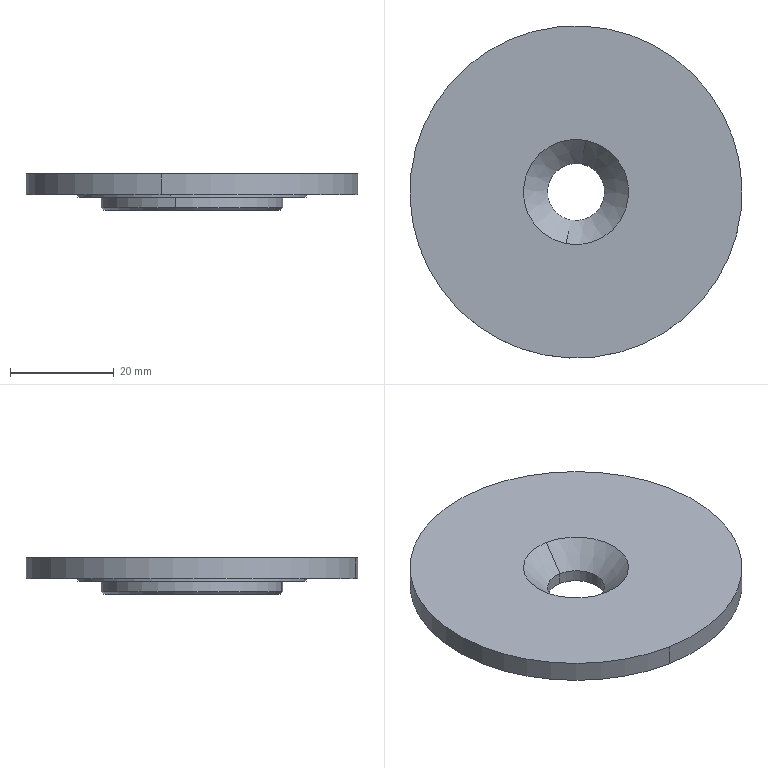Component | SolidWorks | 12AFixedFlatGrooveLargeWheel-EngravingAndMillingAxis-2_12ALargeStraighteningWheelCover-1 | 1 solid | 16 faces | box 64 x 64 x 7 mm | volume 14876 mm3 | cylinder 8 | cone 4 | plane 4 | commonest cylinder face diameters 11 x2 64 x2 44 x2 35 x2 | material 45
build123d program:
from build123d import *

# Parameters (mm, degrees)
HOLE_SIZE_ACCORDING_TO_HEXAGON_SOCKET_D           = 11
HOLE_SIZE_ACCORDING_TO_HEXAGON_SOCKET_DEPTH       = 32.75
HOLE_SIZE_ACCORDING_TO_HEXAGON_SOCKET_CSINK_D     = 20.3
HOLE_SIZE_ACCORDING_TO_HEXAGON_SOCKET_CSINK_ANGLE = 90
HOLE_SIZE_ACCORDING_TO_HEXAGON_SOCKET_TIP         = 3.305
CHAMFER1_SIZE                                     = 0.5


with BuildPart() as part:
    # Sketch1 → Revolve1 (revolve)
    with BuildSketch(Plane.XY, mode=Mode.PRIVATE) as revolve1_sk:
        Polygon((0, 0), (0, 17.5), (2.5, 17.5), (2.5, 22), (3, 22), (3, 32), (7, 32), (7, 0), align=None)
    revolve(revolve1_sk.sketch.rotate(Axis((0, 0, 0), (1, 0, 0)), 90), axis=Axis((0, 0, 0), (1, 0, 0)))

    # Hole Size _ according to_ Hexagon Socket
    with Locations(Plane(origin=(7, 0, 0), x_dir=(0, 0, -1), z_dir=(1, 0, 0))):
        with Locations((0, 0)):
            CounterSinkHole(HOLE_SIZE_ACCORDING_TO_HEXAGON_SOCKET_D / 2, HOLE_SIZE_ACCORDING_TO_HEXAGON_SOCKET_CSINK_D / 2, depth=HOLE_SIZE_ACCORDING_TO_HEXAGON_SOCKET_DEPTH, counter_sink_angle=HOLE_SIZE_ACCORDING_TO_HEXAGON_SOCKET_CSINK_ANGLE)
            with Locations((0, 0, -(HOLE_SIZE_ACCORDING_TO_HEXAGON_SOCKET_DEPTH + HOLE_SIZE_ACCORDING_TO_HEXAGON_SOCKET_TIP / 2))):  # 118° drill point
                Cone(0, HOLE_SIZE_ACCORDING_TO_HEXAGON_SOCKET_D / 2, HOLE_SIZE_ACCORDING_TO_HEXAGON_SOCKET_TIP, mode=Mode.SUBTRACT)

    # Chamfer1
    chamfer1_edges = [part.edges().sort_by_distance(p)[0] for p in [
        (0, 0, -17.5),
    ]]
    chamfer(chamfer1_edges, length=CHAMFER1_SIZE)


solid = part.part

# Placed as in the assembly
solid = solid.moved(Location((-257.402, 59.038, 49.25), (0, -90, 0)))
STEP:
#1=COLOUR_RGB('',0.7922,0.8196,0.9333);
#2=FILL_AREA_STYLE_COLOUR('',#1);
#3=FILL_AREA_STYLE('',(#2));
#4=SURFACE_STYLE_FILL_AREA(#3);
#5=SURFACE_SIDE_STYLE('',(#4));
#6=SURFACE_STYLE_USAGE(.BOTH.,#5);
#7=PRESENTATION_STYLE_ASSIGNMENT((#6));
#8=CARTESIAN_POINT('',(-10.259,1.667,1.939));
#9=VERTEX_POINT('',#8);
#10=CARTESIAN_POINT('',(-10.009,2.982,1.939));
#11=VERTEX_POINT('',#10);
#12=CARTESIAN_POINT('',(-10.134,2.324,1.939));
#13=DIRECTION('',(-0.,0.,-1.));
#14=DIRECTION('',(0.1862,0.9825,0.));
#15=AXIS2_PLACEMENT_3D('',#12,#13,#14);
#16=CIRCLE('',#15,0.6693);
#17=EDGE_CURVE('',#9,#11,#16,.T.);
#18=ORIENTED_EDGE('',*,*,#17,.F.);
#19=CARTESIAN_POINT('',(-10.262,1.647,1.959));
#20=VERTEX_POINT('',#19);
#21=CARTESIAN_POINT('',(-10.259,1.667,1.939));
#22=DIRECTION('',(-0.1316,-0.6947,0.7071));
#23=VECTOR('',#22,39.37);
#24=LINE('',#21,#23);
#25=EDGE_CURVE('',#9,#20,#24,.T.);
#26=ORIENTED_EDGE('',*,*,#25,.T.);
#27=CARTESIAN_POINT('',(-10.006,3.001,1.959));
#28=VERTEX_POINT('',#27);
#29=CARTESIAN_POINT('',(-10.134,2.324,1.959));
#30=DIRECTION('',(0.,-0.,1.));
#31=DIRECTION('',(0.1862,0.9825,0.));
#32=AXIS2_PLACEMENT_3D('',#29,#30,#31);
#33=CIRCLE('',#32,0.689);
#34=EDGE_CURVE('',#28,#20,#33,.T.);
#35=ORIENTED_EDGE('',*,*,#34,.F.);
#36=CARTESIAN_POINT('',(-10.009,2.982,1.939));
#37=DIRECTION('',(0.1316,0.6947,0.7071));
#38=VECTOR('',#37,39.37);
#39=LINE('',#36,#38);
#40=EDGE_CURVE('',#11,#28,#39,.T.);
#41=ORIENTED_EDGE('',*,*,#40,.F.);
#42=EDGE_LOOP('',(#18,#26,#35,#41));
#43=FACE_OUTER_BOUND('',#42,.T.);
#44=CARTESIAN_POINT('',(-10.134,2.324,1.939));
#45=DIRECTION('',(0.,-0.,1.));
#46=DIRECTION('',(0.1862,0.9825,0.));
#47=AXIS2_PLACEMENT_3D('',#44,#45,#46);
#48=CONICAL_SURFACE('',#47,0.6693,0.7854);
#49=ADVANCED_FACE('',(#43),#48,.T.);
#50=CARTESIAN_POINT('',(-10.174,2.112,2.031));
#51=VERTEX_POINT('',#50);
#52=CARTESIAN_POINT('',(-10.094,2.537,2.031));
#53=VERTEX_POINT('',#52);
#54=CARTESIAN_POINT('',(-10.134,2.324,2.031));
#55=DIRECTION('',(0.,-0.,1.));
#56=DIRECTION('',(0.1862,0.9825,0.));
#57=AXIS2_PLACEMENT_3D('',#54,#55,#56);
#58=CIRCLE('',#57,0.2165);
#59=EDGE_CURVE('',#51,#53,#58,.T.);
#60=ORIENTED_EDGE('',*,*,#59,.F.);
#61=CARTESIAN_POINT('',(-10.208,1.932,2.215));
#62=VERTEX_POINT('',#61);
#63=CARTESIAN_POINT('',(-10.208,1.932,2.215));
#64=DIRECTION('',(-0.1316,-0.6947,0.7071));
#65=VECTOR('',#64,39.37);
#66=LINE('',#63,#65);
#67=EDGE_CURVE('',#51,#62,#66,.T.);
#68=ORIENTED_EDGE('',*,*,#67,.T.);
#69=CARTESIAN_POINT('',(-10.06,2.717,2.215));
#70=VERTEX_POINT('',#69);
#71=CARTESIAN_POINT('',(-10.134,2.324,2.215));
#72=DIRECTION('',(0.,-0.,1.));
#73=DIRECTION('',(0.1862,0.9825,0.));
#74=AXIS2_PLACEMENT_3D('',#71,#72,#73);
#75=CIRCLE('',#74,0.3996);
#76=EDGE_CURVE('',#62,#70,#75,.T.);
#77=ORIENTED_EDGE('',*,*,#76,.T.);
#78=CARTESIAN_POINT('',(-10.06,2.717,2.215));
#79=DIRECTION('',(0.1316,0.6947,0.7071));
#80=VECTOR('',#79,39.37);
#81=LINE('',#78,#80);
#82=EDGE_CURVE('',#53,#70,#81,.T.);
#83=ORIENTED_EDGE('',*,*,#82,.F.);
#84=EDGE_LOOP('',(#60,#68,#77,#83));
#85=FACE_OUTER_BOUND('',#84,.T.);
#86=CARTESIAN_POINT('',(-10.134,2.324,2.215));
#87=DIRECTION('',(0.,-0.,1.));
#88=DIRECTION('',(0.1862,0.9825,0.));
#89=AXIS2_PLACEMENT_3D('',#86,#87,#88);
#90=CONICAL_SURFACE('',#89,0.3996,0.7854);
#91=ADVANCED_FACE('',(#85),#90,.F.);
#92=CARTESIAN_POINT('',(-10.174,2.112,1.939));
#93=VERTEX_POINT('',#92);
#94=CARTESIAN_POINT('',(-10.094,2.537,1.939));
#95=VERTEX_POINT('',#94);
#96=CARTESIAN_POINT('',(-10.134,2.324,1.939));
#97=DIRECTION('',(0.,-0.,1.));
#98=DIRECTION('',(0.1862,0.9825,0.));
#99=AXIS2_PLACEMENT_3D('',#96,#97,#98);
#100=CIRCLE('',#99,0.2165);
#101=EDGE_CURVE('',#93,#95,#100,.T.);
#102=ORIENTED_EDGE('',*,*,#101,.F.);
#103=CARTESIAN_POINT('',(-10.174,2.112,2.215));
#104=DIRECTION('',(0.,-0.,1.));
#105=VECTOR('',#104,39.37);
#106=LINE('',#103,#105);
#107=EDGE_CURVE('',#93,#51,#106,.T.);
#108=ORIENTED_EDGE('',*,*,#107,.T.);
#109=ORIENTED_EDGE('',*,*,#59,.T.);
#110=CARTESIAN_POINT('',(-10.094,2.537,2.215));
#111=DIRECTION('',(0.,-0.,1.));
#112=VECTOR('',#111,39.37);
#113=LINE('',#110,#112);
#114=EDGE_CURVE('',#95,#53,#113,.T.);
#115=ORIENTED_EDGE('',*,*,#114,.F.);
#116=EDGE_LOOP('',(#102,#108,#109,#115));
#117=FACE_OUTER_BOUND('',#116,.T.);
#118=CARTESIAN_POINT('',(-10.134,2.324,2.215));
#119=DIRECTION('',(0.,-0.,1.));
#120=DIRECTION('',(0.1862,0.9825,0.));
#121=AXIS2_PLACEMENT_3D('',#118,#119,#120);
#122=CYLINDRICAL_SURFACE('',#121,0.2165);
#123=ADVANCED_FACE('',(#117),#122,.F.);
#124=CARTESIAN_POINT('',(-10.368,1.087,2.215));
#125=VERTEX_POINT('',#124);
#126=CARTESIAN_POINT('',(-9.899,3.562,2.215));
#127=VERTEX_POINT('',#126);
#128=CARTESIAN_POINT('',(-10.134,2.324,2.215));
#129=DIRECTION('',(-0.,0.,-1.));
#130=DIRECTION('',(-0.1862,-0.9825,0.));
#131=AXIS2_PLACEMENT_3D('',#128,#129,#130);
#132=CIRCLE('',#131,1.26);
#133=EDGE_CURVE('',#125,#127,#132,.T.);
#134=ORIENTED_EDGE('',*,*,#133,.T.);
#135=CARTESIAN_POINT('',(-9.899,3.562,2.057));
#136=VERTEX_POINT('',#135);
#137=CARTESIAN_POINT('',(-9.899,3.562,1.939));
#138=DIRECTION('',(-0.,0.,-1.));
#139=VECTOR('',#138,39.37);
#140=LINE('',#137,#139);
#141=EDGE_CURVE('',#127,#136,#140,.T.);
#142=ORIENTED_EDGE('',*,*,#141,.T.);
#143=CARTESIAN_POINT('',(-10.368,1.087,2.057));
#144=VERTEX_POINT('',#143);
#145=CARTESIAN_POINT('',(-10.134,2.324,2.057));
#146=DIRECTION('',(-0.,0.,-1.));
#147=DIRECTION('',(-0.1862,-0.9825,0.));
#148=AXIS2_PLACEMENT_3D('',#145,#146,#147);
#149=CIRCLE('',#148,1.26);
#150=EDGE_CURVE('',#144,#136,#149,.T.);
#151=ORIENTED_EDGE('',*,*,#150,.F.);
#152=CARTESIAN_POINT('',(-10.368,1.087,1.939));
#153=DIRECTION('',(-0.,0.,-1.));
#154=VECTOR('',#153,39.37);
#155=LINE('',#152,#154);
#156=EDGE_CURVE('',#125,#144,#155,.T.);
#157=ORIENTED_EDGE('',*,*,#156,.F.);
#158=EDGE_LOOP('',(#134,#142,#151,#157));
#159=FACE_OUTER_BOUND('',#158,.T.);
#160=CARTESIAN_POINT('',(-10.134,2.324,1.939));
#161=DIRECTION('',(-0.,0.,-1.));
#162=DIRECTION('',(-0.1862,-0.9825,0.));
#163=AXIS2_PLACEMENT_3D('',#160,#161,#162);
#164=CYLINDRICAL_SURFACE('',#163,1.26);
#165=ADVANCED_FACE('',(#159),#164,.T.);
#166=CARTESIAN_POINT('',(-10.295,1.473,2.057));
#167=VERTEX_POINT('',#166);
#168=CARTESIAN_POINT('',(-9.973,3.175,2.057));
#169=VERTEX_POINT('',#168);
#170=CARTESIAN_POINT('',(-10.134,2.324,2.057));
#171=DIRECTION('',(-0.,0.,-1.));
#172=DIRECTION('',(-0.1862,-0.9825,0.));
#173=AXIS2_PLACEMENT_3D('',#170,#171,#172);
#174=CIRCLE('',#173,0.8661);
#175=EDGE_CURVE('',#167,#169,#174,.T.);
#176=ORIENTED_EDGE('',*,*,#175,.T.);
#177=CARTESIAN_POINT('',(-9.973,3.175,2.037));
#178=VERTEX_POINT('',#177);
#179=CARTESIAN_POINT('',(-9.973,3.175,1.939));
#180=DIRECTION('',(-0.,0.,-1.));
#181=VECTOR('',#180,39.37);
#182=LINE('',#179,#181);
#183=EDGE_CURVE('',#169,#178,#182,.T.);
#184=ORIENTED_EDGE('',*,*,#183,.T.);
#185=CARTESIAN_POINT('',(-10.295,1.473,2.037));
#186=VERTEX_POINT('',#185);
#187=CARTESIAN_POINT('',(-10.134,2.324,2.037));
#188=DIRECTION('',(-0.,0.,-1.));
#189=DIRECTION('',(-0.1862,-0.9825,0.));
#190=AXIS2_PLACEMENT_3D('',#187,#188,#189);
#191=CIRCLE('',#190,0.8661);
#192=EDGE_CURVE('',#186,#178,#191,.T.);
#193=ORIENTED_EDGE('',*,*,#192,.F.);
#194=CARTESIAN_POINT('',(-10.295,1.473,1.939));
#195=DIRECTION('',(-0.,0.,-1.));
#196=VECTOR('',#195,39.37);
#197=LINE('',#194,#196);
#198=EDGE_CURVE('',#167,#186,#197,.T.);
#199=ORIENTED_EDGE('',*,*,#198,.F.);
#200=EDGE_LOOP('',(#176,#184,#193,#199));
#201=FACE_OUTER_BOUND('',#200,.T.);
#202=CARTESIAN_POINT('',(-10.134,2.324,1.939));
#203=DIRECTION('',(-0.,0.,-1.));
#204=DIRECTION('',(-0.1862,-0.9825,0.));
#205=AXIS2_PLACEMENT_3D('',#202,#203,#204);
#206=CYLINDRICAL_SURFACE('',#205,0.8661);
#207=ADVANCED_FACE('',(#201),#206,.T.);
#208=CARTESIAN_POINT('',(-10.262,1.647,2.037));
#209=VERTEX_POINT('',#208);
#210=CARTESIAN_POINT('',(-10.006,3.001,2.037));
#211=VERTEX_POINT('',#210);
#212=CARTESIAN_POINT('',(-10.134,2.324,2.037));
#213=DIRECTION('',(-0.,0.,-1.));
#214=DIRECTION('',(-0.1862,-0.9825,0.));
#215=AXIS2_PLACEMENT_3D('',#212,#213,#214);
#216=CIRCLE('',#215,0.689);
#217=EDGE_CURVE('',#209,#211,#216,.T.);
#218=ORIENTED_EDGE('',*,*,#217,.T.);
#219=CARTESIAN_POINT('',(-10.006,3.001,1.939));
#220=DIRECTION('',(-0.,0.,-1.));
#221=VECTOR('',#220,39.37);
#222=LINE('',#219,#221);
#223=EDGE_CURVE('',#211,#28,#222,.T.);
#224=ORIENTED_EDGE('',*,*,#223,.T.);
#225=ORIENTED_EDGE('',*,*,#34,.T.);
#226=CARTESIAN_POINT('',(-10.262,1.647,1.939));
#227=DIRECTION('',(-0.,0.,-1.));
#228=VECTOR('',#227,39.37);
#229=LINE('',#226,#228);
#230=EDGE_CURVE('',#209,#20,#229,.T.);
#231=ORIENTED_EDGE('',*,*,#230,.F.);
#232=EDGE_LOOP('',(#218,#224,#225,#231));
#233=FACE_OUTER_BOUND('',#232,.T.);
#234=CARTESIAN_POINT('',(-10.134,2.324,1.939));
#235=DIRECTION('',(-0.,0.,-1.));
#236=DIRECTION('',(-0.1862,-0.9825,0.));
#237=AXIS2_PLACEMENT_3D('',#234,#235,#236);
#238=CYLINDRICAL_SURFACE('',#237,0.689);
#239=ADVANCED_FACE('',(#233),#238,.T.);
#240=CARTESIAN_POINT('',(-10.134,2.324,1.939));
#241=DIRECTION('',(-0.,0.,-1.));
#242=DIRECTION('',(0.1862,0.9825,0.));
#243=AXIS2_PLACEMENT_3D('',#240,#241,#242);
#244=CIRCLE('',#243,0.6693);
#245=EDGE_CURVE('',#11,#9,#244,.T.);
#246=ORIENTED_EDGE('',*,*,#245,.T.);
#247=ORIENTED_EDGE('',*,*,#17,.T.);
#248=EDGE_LOOP('',(#246,#247));
#249=FACE_OUTER_BOUND('',#248,.T.);
#250=CARTESIAN_POINT('',(-10.134,2.324,1.939));
#251=DIRECTION('',(0.,-0.,1.));
#252=DIRECTION('',(0.1862,0.9825,0.));
#253=AXIS2_PLACEMENT_3D('',#250,#251,#252);
#254=CIRCLE('',#253,0.2165);
#255=EDGE_CURVE('',#95,#93,#254,.T.);
#256=ORIENTED_EDGE('',*,*,#255,.T.);
#257=ORIENTED_EDGE('',*,*,#101,.T.);
#258=EDGE_LOOP('',(#256,#257));
#259=FACE_BOUND('',#258,.T.);
#260=CARTESIAN_POINT('',(-10.134,2.324,1.939));
#261=DIRECTION('',(0.,-0.,1.));
#262=DIRECTION('',(0.1862,0.9825,0.));
#263=AXIS2_PLACEMENT_3D('',#260,#261,#262);
#264=PLANE('',#263);
#265=ADVANCED_FACE('',(#249,#259),#264,.F.);
#266=ORIENTED_EDGE('',*,*,#223,.F.);
#267=CARTESIAN_POINT('',(-10.134,2.324,2.037));
#268=DIRECTION('',(-0.,0.,-1.));
#269=DIRECTION('',(-0.1862,-0.9825,0.));
#270=AXIS2_PLACEMENT_3D('',#267,#268,#269);
#271=CIRCLE('',#270,0.689);
#272=EDGE_CURVE('',#211,#209,#271,.T.);
#273=ORIENTED_EDGE('',*,*,#272,.T.);
#274=ORIENTED_EDGE('',*,*,#230,.T.);
#275=CARTESIAN_POINT('',(-10.134,2.324,1.959));
#276=DIRECTION('',(0.,-0.,1.));
#277=DIRECTION('',(0.1862,0.9825,0.));
#278=AXIS2_PLACEMENT_3D('',#275,#276,#277);
#279=CIRCLE('',#278,0.689);
#280=EDGE_CURVE('',#20,#28,#279,.T.);
#281=ORIENTED_EDGE('',*,*,#280,.T.);
#282=EDGE_LOOP('',(#266,#273,#274,#281));
#283=FACE_OUTER_BOUND('',#282,.T.);
#284=CARTESIAN_POINT('',(-10.134,2.324,1.939));
#285=DIRECTION('',(-0.,0.,-1.));
#286=DIRECTION('',(-0.1862,-0.9825,0.));
#287=AXIS2_PLACEMENT_3D('',#284,#285,#286);
#288=CYLINDRICAL_SURFACE('',#287,0.689);
#289=ADVANCED_FACE('',(#283),#288,.T.);
#290=ORIENTED_EDGE('',*,*,#217,.F.);
#291=ORIENTED_EDGE('',*,*,#272,.F.);
#292=EDGE_LOOP('',(#290,#291));
#293=FACE_BOUND('',#292,.T.);
#294=ORIENTED_EDGE('',*,*,#192,.T.);
#295=CARTESIAN_POINT('',(-10.134,2.324,2.037));
#296=DIRECTION('',(-0.,0.,-1.));
#297=DIRECTION('',(-0.1862,-0.9825,0.));
#298=AXIS2_PLACEMENT_3D('',#295,#296,#297);
#299=CIRCLE('',#298,0.8661);
#300=EDGE_CURVE('',#178,#186,#299,.T.);
#301=ORIENTED_EDGE('',*,*,#300,.T.);
#302=EDGE_LOOP('',(#294,#301));
#303=FACE_OUTER_BOUND('',#302,.T.);
#304=CARTESIAN_POINT('',(-10.811,2.453,2.037));
#305=DIRECTION('',(0.,-0.,1.));
#306=DIRECTION('',(0.1862,0.9825,0.));
#307=AXIS2_PLACEMENT_3D('',#304,#305,#306);
#308=PLANE('',#307);
#309=ADVANCED_FACE('',(#293,#303),#308,.F.);
#310=ORIENTED_EDGE('',*,*,#183,.F.);
#311=CARTESIAN_POINT('',(-10.134,2.324,2.057));
#312=DIRECTION('',(-0.,0.,-1.));
#313=DIRECTION('',(-0.1862,-0.9825,0.));
#314=AXIS2_PLACEMENT_3D('',#311,#312,#313);
#315=CIRCLE('',#314,0.8661);
#316=EDGE_CURVE('',#169,#167,#315,.T.);
#317=ORIENTED_EDGE('',*,*,#316,.T.);
#318=ORIENTED_EDGE('',*,*,#198,.T.);
#319=ORIENTED_EDGE('',*,*,#300,.F.);
#320=EDGE_LOOP('',(#310,#317,#318,#319));
#321=FACE_OUTER_BOUND('',#320,.T.);
#322=CARTESIAN_POINT('',(-10.134,2.324,1.939));
#323=DIRECTION('',(-0.,0.,-1.));
#324=DIRECTION('',(-0.1862,-0.9825,0.));
#325=AXIS2_PLACEMENT_3D('',#322,#323,#324);
#326=CYLINDRICAL_SURFACE('',#325,0.8661);
#327=ADVANCED_FACE('',(#321),#326,.T.);
#328=ORIENTED_EDGE('',*,*,#175,.F.);
#329=ORIENTED_EDGE('',*,*,#316,.F.);
#330=EDGE_LOOP('',(#328,#329));
#331=FACE_BOUND('',#330,.T.);
#332=ORIENTED_EDGE('',*,*,#150,.T.);
#333=CARTESIAN_POINT('',(-10.134,2.324,2.057));
#334=DIRECTION('',(-0.,0.,-1.));
#335=DIRECTION('',(-0.1862,-0.9825,0.));
#336=AXIS2_PLACEMENT_3D('',#333,#334,#335);
#337=CIRCLE('',#336,1.26);
#338=EDGE_CURVE('',#136,#144,#337,.T.);
#339=ORIENTED_EDGE('',*,*,#338,.T.);
#340=EDGE_LOOP('',(#332,#339));
#341=FACE_OUTER_BOUND('',#340,.T.);
#342=CARTESIAN_POINT('',(-10.985,2.486,2.057));
#343=DIRECTION('',(0.,-0.,1.));
#344=DIRECTION('',(0.1862,0.9825,0.));
#345=AXIS2_PLACEMENT_3D('',#342,#343,#344);
#346=PLANE('',#345);
#347=ADVANCED_FACE('',(#331,#341),#346,.F.);
#348=ORIENTED_EDGE('',*,*,#141,.F.);
#349=CARTESIAN_POINT('',(-10.134,2.324,2.215));
#350=DIRECTION('',(-0.,0.,-1.));
#351=DIRECTION('',(-0.1862,-0.9825,0.));
#352=AXIS2_PLACEMENT_3D('',#349,#350,#351);
#353=CIRCLE('',#352,1.26);
#354=EDGE_CURVE('',#127,#125,#353,.T.);
#355=ORIENTED_EDGE('',*,*,#354,.T.);
#356=ORIENTED_EDGE('',*,*,#156,.T.);
#357=ORIENTED_EDGE('',*,*,#338,.F.);
#358=EDGE_LOOP('',(#348,#355,#356,#357));
#359=FACE_OUTER_BOUND('',#358,.T.);
#360=CARTESIAN_POINT('',(-10.134,2.324,1.939));
#361=DIRECTION('',(-0.,0.,-1.));
#362=DIRECTION('',(-0.1862,-0.9825,0.));
#363=AXIS2_PLACEMENT_3D('',#360,#361,#362);
#364=CYLINDRICAL_SURFACE('',#363,1.26);
#365=ADVANCED_FACE('',(#359),#364,.T.);
#366=CARTESIAN_POINT('',(-10.134,2.324,2.215));
#367=DIRECTION('',(0.,-0.,1.));
#368=DIRECTION('',(0.1862,0.9825,0.));
#369=AXIS2_PLACEMENT_3D('',#366,#367,#368);
#370=CIRCLE('',#369,0.3996);
#371=EDGE_CURVE('',#70,#62,#370,.T.);
#372=ORIENTED_EDGE('',*,*,#371,.F.);
#373=ORIENTED_EDGE('',*,*,#76,.F.);
#374=EDGE_LOOP('',(#372,#373));
#375=FACE_BOUND('',#374,.T.);
#376=ORIENTED_EDGE('',*,*,#133,.F.);
#377=ORIENTED_EDGE('',*,*,#354,.F.);
#378=EDGE_LOOP('',(#376,#377));
#379=FACE_OUTER_BOUND('',#378,.T.);
#380=CARTESIAN_POINT('',(-11.372,2.559,2.215));
#381=DIRECTION('',(-0.,0.,-1.));
#382=DIRECTION('',(-0.1862,-0.9825,-0.));
#383=AXIS2_PLACEMENT_3D('',#380,#381,#382);
#384=PLANE('',#383);
#385=ADVANCED_FACE('',(#375,#379),#384,.F.);
#386=ORIENTED_EDGE('',*,*,#107,.F.);
#387=ORIENTED_EDGE('',*,*,#255,.F.);
#388=ORIENTED_EDGE('',*,*,#114,.T.);
#389=CARTESIAN_POINT('',(-10.134,2.324,2.031));
#390=DIRECTION('',(0.,-0.,1.));
#391=DIRECTION('',(0.1862,0.9825,0.));
#392=AXIS2_PLACEMENT_3D('',#389,#390,#391);
#393=CIRCLE('',#392,0.2165);
#394=EDGE_CURVE('',#53,#51,#393,.T.);
#395=ORIENTED_EDGE('',*,*,#394,.T.);
#396=EDGE_LOOP('',(#386,#387,#388,#395));
#397=FACE_OUTER_BOUND('',#396,.T.);
#398=CARTESIAN_POINT('',(-10.134,2.324,2.215));
#399=DIRECTION('',(0.,-0.,1.));
#400=DIRECTION('',(0.1862,0.9825,0.));
#401=AXIS2_PLACEMENT_3D('',#398,#399,#400);
#402=CYLINDRICAL_SURFACE('',#401,0.2165);
#403=ADVANCED_FACE('',(#397),#402,.F.);
#404=ORIENTED_EDGE('',*,*,#67,.F.);
#405=ORIENTED_EDGE('',*,*,#394,.F.);
#406=ORIENTED_EDGE('',*,*,#82,.T.);
#407=ORIENTED_EDGE('',*,*,#371,.T.);
#408=EDGE_LOOP('',(#404,#405,#406,#407));
#409=FACE_OUTER_BOUND('',#408,.T.);
#410=CARTESIAN_POINT('',(-10.134,2.324,2.215));
#411=DIRECTION('',(0.,-0.,1.));
#412=DIRECTION('',(0.1862,0.9825,0.));
#413=AXIS2_PLACEMENT_3D('',#410,#411,#412);
#414=CONICAL_SURFACE('',#413,0.3996,0.7854);
#415=ADVANCED_FACE('',(#409),#414,.F.);
#416=ORIENTED_EDGE('',*,*,#25,.F.);
#417=ORIENTED_EDGE('',*,*,#245,.F.);
#418=ORIENTED_EDGE('',*,*,#40,.T.);
#419=ORIENTED_EDGE('',*,*,#280,.F.);
#420=EDGE_LOOP('',(#416,#417,#418,#419));
#421=FACE_OUTER_BOUND('',#420,.T.);
#422=CARTESIAN_POINT('',(-10.134,2.324,1.939));
#423=DIRECTION('',(0.,-0.,1.));
#424=DIRECTION('',(0.1862,0.9825,0.));
#425=AXIS2_PLACEMENT_3D('',#422,#423,#424);
#426=CONICAL_SURFACE('',#425,0.6693,0.7854);
#427=ADVANCED_FACE('',(#421),#426,.T.);
#428=CLOSED_SHELL('',(#49,#91,#123,#165,#207,#239,#265,#289,#309,#327,#347,#365,#385,#403,#415,#427));
#429=MANIFOLD_SOLID_BREP('',#428);
#430=STYLED_ITEM('',(#7),#429);
#431=PRESENTATION_LAYER_ASSIGNMENT('','',(#430));
#432=CARTESIAN_POINT('',(0.,0.,0.));
#433=DIRECTION('',(0.,0.,1.));
#434=DIRECTION('',(1.,0.,0.));
#435=AXIS2_PLACEMENT_3D('',#432,#433,#434);
#436=(LENGTH_UNIT()NAMED_UNIT(*)SI_UNIT($,.METRE.));
#437=LENGTH_MEASURE_WITH_UNIT(LENGTH_MEASURE(0.0254),#436);
#438=DIMENSIONAL_EXPONENTS(1.,0.,0.,0.,0.,0.,0.);
#439=(CONVERSION_BASED_UNIT('',#437)LENGTH_UNIT()NAMED_UNIT(#438));
#440=UNCERTAINTY_MEASURE_WITH_UNIT(LENGTH_MEASURE(0.00001),#439,'','');
#441=(NAMED_UNIT(*)PLANE_ANGLE_UNIT()SI_UNIT($,.RADIAN.));
#442=(NAMED_UNIT(*)SI_UNIT($,.STERADIAN.)SOLID_ANGLE_UNIT());
#443=(GEOMETRIC_REPRESENTATION_CONTEXT(3)GLOBAL_UNCERTAINTY_ASSIGNED_CONTEXT((#440))GLOBAL_UNIT_ASSIGNED_CONTEXT((#439,#441,#442))REPRESENTATION_CONTEXT('',''));
#444=ADVANCED_BREP_SHAPE_REPRESENTATION('',(#429,#435),#443);
#445=(LENGTH_UNIT()NAMED_UNIT(*)SI_UNIT($,.METRE.));
#446=LENGTH_MEASURE_WITH_UNIT(LENGTH_MEASURE(0.0254),#445);
#447=DIMENSIONAL_EXPONENTS(1.,0.,0.,0.,0.,0.,0.);
#448=(CONVERSION_BASED_UNIT('',#446)LENGTH_UNIT()NAMED_UNIT(#447));
#449=UNCERTAINTY_MEASURE_WITH_UNIT(LENGTH_MEASURE(0.00001),#448,'','');
#450=(NAMED_UNIT(*)PLANE_ANGLE_UNIT()SI_UNIT($,.RADIAN.));
#451=(NAMED_UNIT(*)SI_UNIT($,.STERADIAN.)SOLID_ANGLE_UNIT());
#452=(GEOMETRIC_REPRESENTATION_CONTEXT(3)GLOBAL_UNCERTAINTY_ASSIGNED_CONTEXT((#449))GLOBAL_UNIT_ASSIGNED_CONTEXT((#448,#450,#451))REPRESENTATION_CONTEXT('',''));
#453=MECHANICAL_DESIGN_GEOMETRIC_PRESENTATION_REPRESENTATION('',(#430),#452);